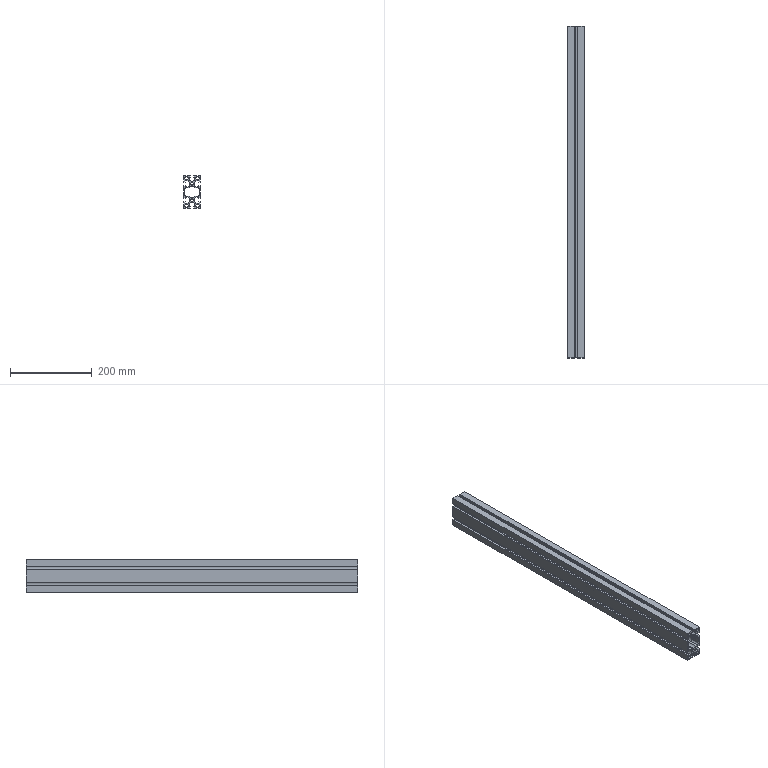Component | SolidWorks | 30-01A-1_EF4080-550-1 | 1 solid | 84 faces | box 40 x 810 x 80 mm | volume 932347 mm3 | plane 58 | cylinder 26 | commonest cylinder face diameters 8 x12 19 x10 6.8 x4
build123d program:
from build123d import *

# Parameters (mm, degrees)
SKETCH1_R      = 4
SKETCH1_R_2    = 3.4
EXTRUDE1_DEPTH = 405


with BuildPart() as part:
    # Sketch1 → Extrude1 (new, symmetric)
    with BuildSketch(Plane(origin=(0, 0, 0), x_dir=(0, 0, -1), z_dir=(0, 1, 0))):
        with BuildLine():
            Line((-40, 20), (-24.2, 20))
            Line((-24.2, 20), (-24.2, 16))
            Line((-24.2, 16), (-27.25, 16))
            Line((-27.25, 16), (-27.25, 9.361))
            ThreePointArc((-27.25, 9.361), (-20, 6), (-12.75, 9.361))
            Line((-12.75, 9.361), (-12.75, 16))
            Line((-12.75, 16), (-15.8, 16))
            Line((-15.8, 16), (-15.8, 20))
            Line((-15.8, 20), (15.8, 20))
            Line((15.8, 20), (15.8, 16))
            Line((15.8, 16), (12.75, 16))
            Line((12.75, 16), (12.75, 9.361))
            ThreePointArc((12.75, 9.361), (20, 6), (27.25, 9.361))
            Line((27.25, 9.361), (27.25, 16))
            Line((27.25, 16), (24.2, 16))
            Line((24.2, 16), (24.2, 20))
            Line((24.2, 20), (40, 20))
            Line((40, 20), (40, 4.2))
            Line((40, 4.2), (36, 4.2))
            Line((36, 4.2), (36, 7.25))
            Line((36, 7.25), (29.361, 7.25))
            ThreePointArc((29.361, 7.25), (26, 0), (29.361, -7.25))
            Line((29.361, -7.25), (36, -7.25))
            Line((36, -7.25), (36, -4.2))
            Line((36, -4.2), (40, -4.2))
            Line((40, -4.2), (40, -20))
            Line((40, -20), (24.2, -20))
            Line((24.2, -20), (24.2, -16))
            Line((24.2, -16), (27.25, -16))
            Line((27.25, -16), (27.25, -9.361))
            ThreePointArc((27.25, -9.361), (20, -6), (12.75, -9.361))
            Line((12.75, -9.361), (12.75, -16))
            Line((12.75, -16), (15.8, -16))
            Line((15.8, -16), (15.8, -20))
            Line((15.8, -20), (-15.8, -20))
            Line((-15.8, -20), (-15.8, -16))
            Line((-15.8, -16), (-12.75, -16))
            Line((-12.75, -16), (-12.75, -9.361))
            ThreePointArc((-12.75, -9.361), (-20, -6), (-27.25, -9.361))
            Line((-27.25, -9.361), (-27.25, -16))
            Line((-27.25, -16), (-24.2, -16))
            Line((-24.2, -16), (-24.2, -20))
            Line((-24.2, -20), (-40, -20))
            Line((-40, -20), (-40, -4.2))
            Line((-40, -4.2), (-36, -4.2))
            Line((-36, -4.2), (-36, -7.25))
            Line((-36, -7.25), (-29.361, -7.25))
            ThreePointArc((-29.361, -7.25), (-26, 0), (-29.361, 7.25))
            Line((-29.361, 7.25), (-36, 7.25))
            Line((-36, 7.25), (-36, 4.2))
            Line((-36, 4.2), (-40, 4.2))
            Line((-40, 4.2), (-40, 20))
        make_face()
        with Locations(Location((-33.5, 13.5, 0), (0, 0, 180))):
            Circle(SKETCH1_R, mode=Mode.SUBTRACT)
        with Locations(Location((-20, 0, 0), (0, 0, 180))):
            Circle(SKETCH1_R_2, mode=Mode.SUBTRACT)
        with Locations((-33.5, -13.5)):
            Circle(SKETCH1_R, mode=Mode.SUBTRACT)
        with Locations(Location((33.5, -13.5, 0), (0, 0, 180))):
            Circle(SKETCH1_R, mode=Mode.SUBTRACT)
        with Locations((20, 0)):
            Circle(SKETCH1_R_2, mode=Mode.SUBTRACT)
        with Locations((33.5, 13.5)):
            Circle(SKETCH1_R, mode=Mode.SUBTRACT)
        with BuildLine():
            Line((-10.5, -7.25), (-10.5, -13.5))
            ThreePointArc((-10.5, -13.5), (-9.328, -16.328), (-6.5, -17.5))
            Line((-6.5, -17.5), (6.5, -17.5))
            ThreePointArc((6.5, -17.5), (9.328, -16.328), (10.5, -13.5))
            Line((10.5, -13.5), (10.5, -7.25))
            Line((10.5, -7.25), (10.639, -7.25))
            ThreePointArc((10.639, -7.25), (14, 0), (10.639, 7.25))
            Line((10.639, 7.25), (10.5, 7.25))
            Line((10.5, 7.25), (10.5, 13.5))
            ThreePointArc((10.5, 13.5), (9.328, 16.328), (6.5, 17.5))
            Line((6.5, 17.5), (-6.5, 17.5))
            ThreePointArc((-6.5, 17.5), (-9.328, 16.328), (-10.5, 13.5))
            Line((-10.5, 13.5), (-10.5, 7.25))
            Line((-10.5, 7.25), (-10.639, 7.25))
            ThreePointArc((-10.639, 7.25), (-14, 0), (-10.639, -7.25))
            Line((-10.639, -7.25), (-10.5, -7.25))
        make_face(mode=Mode.SUBTRACT)
    extrude(amount=EXTRUDE1_DEPTH, both=True)


solid = part.part

# Placed as in the assembly
solid = solid.moved(Location((-427.43, -52.845, -970), (0, 0, 0)))